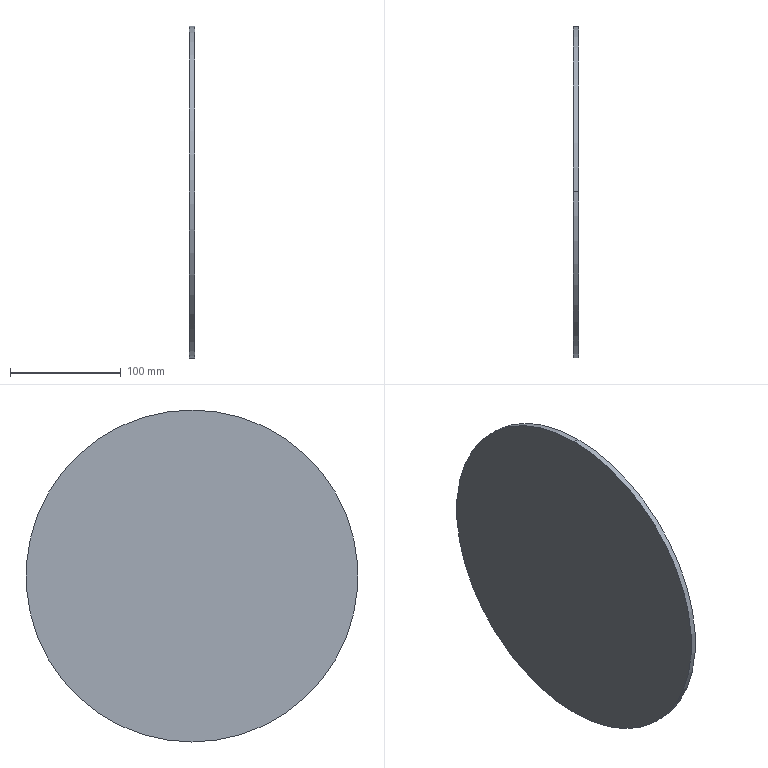Component | SolidWorks | JF21-80.1-1-3(_)-1-SOLID4-1 | 1 solid | 4 faces | box 5 x 300 x 300 mm | volume 353429 mm3 | cylinder 2 | plane 2 | commonest cylinder face diameters 300 x2
STEP:
#1=CARTESIAN_POINT('',(5.315,-39.37,42.126));
#2=VERTEX_POINT('',#1);
#3=CARTESIAN_POINT('',(5.315,-39.37,30.315));
#4=VERTEX_POINT('',#3);
#5=CARTESIAN_POINT('',(5.315,-39.37,36.22));
#6=DIRECTION('',(-1.,0.,0.));
#7=DIRECTION('',(0.,0.,1.));
#8=AXIS2_PLACEMENT_3D('',#5,#6,#7);
#9=CIRCLE('',#8,5.906);
#10=EDGE_CURVE('',#2,#4,#9,.T.);
#11=ORIENTED_EDGE('',*,*,#10,.F.);
#12=CARTESIAN_POINT('',(5.512,-39.37,42.126));
#13=VERTEX_POINT('',#12);
#14=CARTESIAN_POINT('',(5.315,-39.37,42.126));
#15=DIRECTION('',(-1.,0.,0.));
#16=VECTOR('',#15,39.37);
#17=LINE('',#14,#16);
#18=EDGE_CURVE('',#13,#2,#17,.T.);
#19=ORIENTED_EDGE('',*,*,#18,.F.);
#20=CARTESIAN_POINT('',(5.512,-39.37,30.315));
#21=VERTEX_POINT('',#20);
#22=CARTESIAN_POINT('',(5.512,-39.37,36.22));
#23=DIRECTION('',(-1.,0.,0.));
#24=DIRECTION('',(0.,0.,1.));
#25=AXIS2_PLACEMENT_3D('',#22,#23,#24);
#26=CIRCLE('',#25,5.906);
#27=EDGE_CURVE('',#13,#21,#26,.T.);
#28=ORIENTED_EDGE('',*,*,#27,.T.);
#29=CARTESIAN_POINT('',(5.315,-39.37,30.315));
#30=DIRECTION('',(-1.,0.,0.));
#31=VECTOR('',#30,39.37);
#32=LINE('',#29,#31);
#33=EDGE_CURVE('',#21,#4,#32,.T.);
#34=ORIENTED_EDGE('',*,*,#33,.T.);
#35=EDGE_LOOP('',(#11,#19,#28,#34));
#36=FACE_OUTER_BOUND('',#35,.T.);
#37=CARTESIAN_POINT('',(5.315,-39.37,36.22));
#38=DIRECTION('',(1.,0.,0.));
#39=DIRECTION('',(0.,0.,1.));
#40=AXIS2_PLACEMENT_3D('',#37,#38,#39);
#41=CYLINDRICAL_SURFACE('',#40,5.906);
#42=ADVANCED_FACE('',(#36),#41,.T.);
#43=ORIENTED_EDGE('',*,*,#18,.T.);
#44=CARTESIAN_POINT('',(5.315,-39.37,36.22));
#45=DIRECTION('',(-1.,0.,0.));
#46=DIRECTION('',(0.,0.,1.));
#47=AXIS2_PLACEMENT_3D('',#44,#45,#46);
#48=CIRCLE('',#47,5.906);
#49=EDGE_CURVE('',#4,#2,#48,.T.);
#50=ORIENTED_EDGE('',*,*,#49,.F.);
#51=ORIENTED_EDGE('',*,*,#33,.F.);
#52=CARTESIAN_POINT('',(5.512,-39.37,36.22));
#53=DIRECTION('',(-1.,0.,0.));
#54=DIRECTION('',(0.,0.,1.));
#55=AXIS2_PLACEMENT_3D('',#52,#53,#54);
#56=CIRCLE('',#55,5.906);
#57=EDGE_CURVE('',#21,#13,#56,.T.);
#58=ORIENTED_EDGE('',*,*,#57,.T.);
#59=EDGE_LOOP('',(#43,#50,#51,#58));
#60=FACE_OUTER_BOUND('',#59,.T.);
#61=CARTESIAN_POINT('',(5.315,-39.37,36.22));
#62=DIRECTION('',(1.,0.,0.));
#63=DIRECTION('',(0.,0.,1.));
#64=AXIS2_PLACEMENT_3D('',#61,#62,#63);
#65=CYLINDRICAL_SURFACE('',#64,5.906);
#66=ADVANCED_FACE('',(#60),#65,.T.);
#67=ORIENTED_EDGE('',*,*,#49,.T.);
#68=ORIENTED_EDGE('',*,*,#10,.T.);
#69=EDGE_LOOP('',(#67,#68));
#70=FACE_OUTER_BOUND('',#69,.T.);
#71=CARTESIAN_POINT('',(5.315,-39.37,36.22));
#72=DIRECTION('',(-1.,0.,0.));
#73=DIRECTION('',(0.,0.,-1.));
#74=AXIS2_PLACEMENT_3D('',#71,#72,#73);
#75=PLANE('',#74);
#76=ADVANCED_FACE('',(#70),#75,.T.);
#77=ORIENTED_EDGE('',*,*,#57,.F.);
#78=ORIENTED_EDGE('',*,*,#27,.F.);
#79=EDGE_LOOP('',(#77,#78));
#80=FACE_OUTER_BOUND('',#79,.T.);
#81=CARTESIAN_POINT('',(5.512,-39.37,36.22));
#82=DIRECTION('',(-1.,0.,0.));
#83=DIRECTION('',(0.,0.,-1.));
#84=AXIS2_PLACEMENT_3D('',#81,#82,#83);
#85=PLANE('',#84);
#86=ADVANCED_FACE('',(#80),#85,.F.);
#87=CLOSED_SHELL('',(#42,#66,#76,#86));
#88=MANIFOLD_SOLID_BREP('',#87);
#89=CARTESIAN_POINT('',(0.,0.,0.));
#90=DIRECTION('',(0.,0.,1.));
#91=DIRECTION('',(1.,0.,0.));
#92=AXIS2_PLACEMENT_3D('',#89,#90,#91);
#93=(LENGTH_UNIT()NAMED_UNIT(*)SI_UNIT($,.METRE.));
#94=LENGTH_MEASURE_WITH_UNIT(LENGTH_MEASURE(0.0254),#93);
#95=DIMENSIONAL_EXPONENTS(1.,0.,0.,0.,0.,0.,0.);
#96=(CONVERSION_BASED_UNIT('',#94)LENGTH_UNIT()NAMED_UNIT(#95));
#97=UNCERTAINTY_MEASURE_WITH_UNIT(LENGTH_MEASURE(0.00001),#96,'','');
#98=(NAMED_UNIT(*)PLANE_ANGLE_UNIT()SI_UNIT($,.RADIAN.));
#99=(NAMED_UNIT(*)SI_UNIT($,.STERADIAN.)SOLID_ANGLE_UNIT());
#100=(GEOMETRIC_REPRESENTATION_CONTEXT(3)GLOBAL_UNCERTAINTY_ASSIGNED_CONTEXT((#97))GLOBAL_UNIT_ASSIGNED_CONTEXT((#96,#98,#99))REPRESENTATION_CONTEXT('',''));
#101=ADVANCED_BREP_SHAPE_REPRESENTATION('',(#88,#92),#100);
#102=COLOUR_RGB('',0.7922,0.8196,0.9333);
#103=FILL_AREA_STYLE_COLOUR('',#102);
#104=FILL_AREA_STYLE('',(#103));
#105=SURFACE_STYLE_FILL_AREA(#104);
#106=SURFACE_SIDE_STYLE('',(#105));
#107=SURFACE_STYLE_USAGE(.BOTH.,#106);
#108=PRESENTATION_STYLE_ASSIGNMENT((#107));
#109=STYLED_ITEM('',(#108),#88);
#110=(LENGTH_UNIT()NAMED_UNIT(*)SI_UNIT($,.METRE.));
#111=LENGTH_MEASURE_WITH_UNIT(LENGTH_MEASURE(0.0254),#110);
#112=DIMENSIONAL_EXPONENTS(1.,0.,0.,0.,0.,0.,0.);
#113=(CONVERSION_BASED_UNIT('',#111)LENGTH_UNIT()NAMED_UNIT(#112));
#114=UNCERTAINTY_MEASURE_WITH_UNIT(LENGTH_MEASURE(0.00001),#113,'','');
#115=(NAMED_UNIT(*)PLANE_ANGLE_UNIT()SI_UNIT($,.RADIAN.));
#116=(NAMED_UNIT(*)SI_UNIT($,.STERADIAN.)SOLID_ANGLE_UNIT());
#117=(GEOMETRIC_REPRESENTATION_CONTEXT(3)GLOBAL_UNCERTAINTY_ASSIGNED_CONTEXT((#114))GLOBAL_UNIT_ASSIGNED_CONTEXT((#113,#115,#116))REPRESENTATION_CONTEXT('',''));
#118=MECHANICAL_DESIGN_GEOMETRIC_PRESENTATION_REPRESENTATION('',(#109),#117);
#119=PRESENTATION_LAYER_ASSIGNMENT('','',(#109));